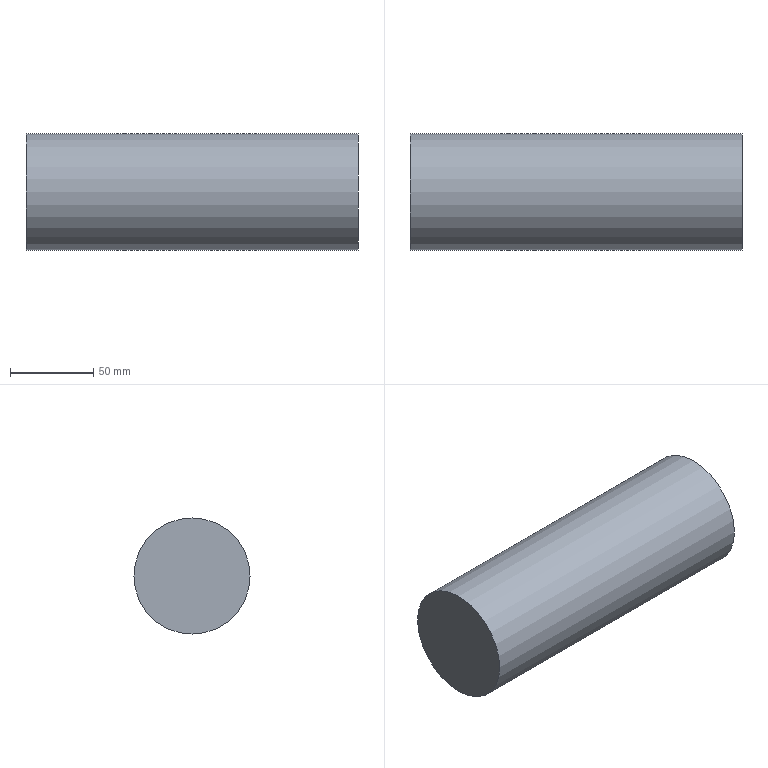Component | NX | SHAFT_PIN_70_200_2 | 1 solid | 3 faces | box 200 x 70 x 70 mm | volume 769690 mm3 | plane 2 | cylinder 1 | commonest cylinder face diameters 70 x1
STEP:
#1=CARTESIAN_POINT('',(0.,0.,0.));
#2=DIRECTION('',(0.,0.,1.));
#3=DIRECTION('',(1.,0.,0.));
#4=AXIS2_PLACEMENT_3D('',#1,#2,#3);
#5=CARTESIAN_POINT('',(-217.564,-1271.553,-235.));
#6=VERTEX_POINT('',#5);
#7=CARTESIAN_POINT('',(-217.564,-1271.553,-200.));
#8=DIRECTION('',(-1.,0.,0.));
#9=DIRECTION('',(0.,0.,-1.));
#10=AXIS2_PLACEMENT_3D('',#7,#8,#9);
#11=CIRCLE('',#10,35.);
#12=CARTESIAN_POINT('',(-217.564,-1271.553,-200.));
#13=DIRECTION('',(1.,0.,0.));
#14=DIRECTION('',(0.,0.,-1.));
#15=AXIS2_PLACEMENT_3D('',#12,#13,#14);
#16=PLANE('',#15);
#17=CARTESIAN_POINT('',(35.,0.));
#18=CARTESIAN_POINT('',(35.,-60.622));
#19=CARTESIAN_POINT('',(-17.5,-30.311));
#20=CARTESIAN_POINT('',(-70.,-0.));
#21=CARTESIAN_POINT('',(-17.5,30.311));
#22=CARTESIAN_POINT('',(35.,60.622));
#23=CARTESIAN_POINT('',(35.,0.));
#24=(BOUNDED_CURVE()B_SPLINE_CURVE(2,(#17,#18,#19,#20,#21,#22,#23),.UNSPECIFIED.,.T.,.F.)B_SPLINE_CURVE_WITH_KNOTS((1,2,2,2,2,1),(-2.094,0.,2.094,4.189,6.283,8.378),.UNSPECIFIED.)CURVE()GEOMETRIC_REPRESENTATION_ITEM()RATIONAL_B_SPLINE_CURVE((1.,0.5,1.,0.5,1.,0.5,1.))REPRESENTATION_ITEM(''));
#25=(GEOMETRIC_REPRESENTATION_CONTEXT(2)PARAMETRIC_REPRESENTATION_CONTEXT()REPRESENTATION_CONTEXT('',''));
#26=DEFINITIONAL_REPRESENTATION('',(#24),#25);
#27=PCURVE('',#16,#26);
#28=CARTESIAN_POINT('',(-417.564,-1271.553,-200.));
#29=DIRECTION('',(1.,0.,0.));
#30=DIRECTION('',(0.,0.,-1.));
#31=AXIS2_PLACEMENT_3D('',#28,#29,#30);
#32=CYLINDRICAL_SURFACE('',#31,35.);
#33=CARTESIAN_POINT('',(6.283,200.));
#34=DIRECTION('',(-1.,0.));
#35=VECTOR('',#34,1.);
#36=LINE('',#33,#35);
#37=(GEOMETRIC_REPRESENTATION_CONTEXT(2)PARAMETRIC_REPRESENTATION_CONTEXT()REPRESENTATION_CONTEXT('',''));
#38=DEFINITIONAL_REPRESENTATION('',(#36),#37);
#39=PCURVE('',#32,#38);
#40=SURFACE_CURVE('',#11,(#27,#39),.PCURVE_S1.);
#41=EDGE_CURVE('',#6,#6,#40,.T.);
#42=ORIENTED_EDGE('',*,*,#41,.F.);
#43=EDGE_LOOP('',(#42));
#44=FACE_BOUND('',#43,.T.);
#45=ADVANCED_FACE('',(#44),#16,.T.);
#46=CARTESIAN_POINT('',(-417.564,-1271.553,-235.));
#47=VERTEX_POINT('',#46);
#48=CARTESIAN_POINT('',(-417.564,-1271.553,-200.));
#49=DIRECTION('',(1.,0.,0.));
#50=DIRECTION('',(0.,0.,-1.));
#51=AXIS2_PLACEMENT_3D('',#48,#49,#50);
#52=CIRCLE('',#51,35.);
#53=CARTESIAN_POINT('',(-417.564,-1271.553,-200.));
#54=DIRECTION('',(-1.,0.,0.));
#55=DIRECTION('',(0.,0.,1.));
#56=AXIS2_PLACEMENT_3D('',#53,#54,#55);
#57=PLANE('',#56);
#58=CARTESIAN_POINT('',(-35.,0.));
#59=CARTESIAN_POINT('',(-35.,60.622));
#60=CARTESIAN_POINT('',(17.5,30.311));
#61=CARTESIAN_POINT('',(70.,0.));
#62=CARTESIAN_POINT('',(17.5,-30.311));
#63=CARTESIAN_POINT('',(-35.,-60.622));
#64=CARTESIAN_POINT('',(-35.,0.));
#65=(BOUNDED_CURVE()B_SPLINE_CURVE(2,(#58,#59,#60,#61,#62,#63,#64),.UNSPECIFIED.,.T.,.F.)B_SPLINE_CURVE_WITH_KNOTS((1,2,2,2,2,1),(-2.094,0.,2.094,4.189,6.283,8.378),.UNSPECIFIED.)CURVE()GEOMETRIC_REPRESENTATION_ITEM()RATIONAL_B_SPLINE_CURVE((1.,0.5,1.,0.5,1.,0.5,1.))REPRESENTATION_ITEM(''));
#66=(GEOMETRIC_REPRESENTATION_CONTEXT(2)PARAMETRIC_REPRESENTATION_CONTEXT()REPRESENTATION_CONTEXT('',''));
#67=DEFINITIONAL_REPRESENTATION('',(#65),#66);
#68=PCURVE('',#57,#67);
#69=CARTESIAN_POINT('',(0.,0.));
#70=DIRECTION('',(1.,0.));
#71=VECTOR('',#70,1.);
#72=LINE('',#69,#71);
#73=(GEOMETRIC_REPRESENTATION_CONTEXT(2)PARAMETRIC_REPRESENTATION_CONTEXT()REPRESENTATION_CONTEXT('',''));
#74=DEFINITIONAL_REPRESENTATION('',(#72),#73);
#75=PCURVE('',#32,#74);
#76=SURFACE_CURVE('',#52,(#68,#75),.PCURVE_S1.);
#77=EDGE_CURVE('',#47,#47,#76,.T.);
#78=ORIENTED_EDGE('',*,*,#77,.F.);
#79=EDGE_LOOP('',(#78));
#80=FACE_BOUND('',#79,.T.);
#81=ADVANCED_FACE('',(#80),#57,.T.);
#82=ORIENTED_EDGE('',*,*,#41,.T.);
#83=CARTESIAN_POINT('',(-417.564,-1271.553,-235.));
#84=CARTESIAN_POINT('',(-217.564,-1271.553,-235.));
#85=B_SPLINE_CURVE_WITH_KNOTS('',1,(#83,#84),.UNSPECIFIED.,.F.,.F.,(2,2),(0.,200.),.PIECEWISE_BEZIER_KNOTS.);
#86=CARTESIAN_POINT('',(0.,0.));
#87=DIRECTION('',(0.,1.));
#88=VECTOR('',#87,1.);
#89=LINE('',#86,#88);
#90=(GEOMETRIC_REPRESENTATION_CONTEXT(2)PARAMETRIC_REPRESENTATION_CONTEXT()REPRESENTATION_CONTEXT('',''));
#91=DEFINITIONAL_REPRESENTATION('',(#89),#90);
#92=PCURVE('',#32,#91);
#93=CARTESIAN_POINT('',(6.283,0.));
#94=DIRECTION('',(0.,1.));
#95=VECTOR('',#94,1.);
#96=LINE('',#93,#95);
#97=(GEOMETRIC_REPRESENTATION_CONTEXT(2)PARAMETRIC_REPRESENTATION_CONTEXT()REPRESENTATION_CONTEXT('',''));
#98=DEFINITIONAL_REPRESENTATION('',(#96),#97);
#99=PCURVE('',#32,#98);
#100=SEAM_CURVE('',#85,(#92,#99),.PCURVE_S1.);
#101=EDGE_CURVE('',#47,#6,#100,.T.);
#102=ORIENTED_EDGE('',*,*,#101,.F.);
#103=ORIENTED_EDGE('',*,*,#77,.T.);
#104=ORIENTED_EDGE('',*,*,#101,.T.);
#105=EDGE_LOOP('',(#82,#102,#103,#104));
#106=FACE_BOUND('',#105,.T.);
#107=ADVANCED_FACE('',(#106),#32,.T.);
#108=CLOSED_SHELL('',(#45,#81,#107));
#109=MANIFOLD_SOLID_BREP('',#108);
#110=(LENGTH_UNIT()NAMED_UNIT(*)SI_UNIT(.MILLI.,.METRE.));
#111=UNCERTAINTY_MEASURE_WITH_UNIT(LENGTH_MEASURE(0.00001),#110,'','');
#112=(NAMED_UNIT(*)PLANE_ANGLE_UNIT()SI_UNIT($,.RADIAN.));
#113=(NAMED_UNIT(*)SI_UNIT($,.STERADIAN.)SOLID_ANGLE_UNIT());
#114=(GEOMETRIC_REPRESENTATION_CONTEXT(3)GLOBAL_UNCERTAINTY_ASSIGNED_CONTEXT((#111))GLOBAL_UNIT_ASSIGNED_CONTEXT((#110,#112,#113))REPRESENTATION_CONTEXT('',''));
#115=ADVANCED_BREP_SHAPE_REPRESENTATION('',(#4,#109),#114);